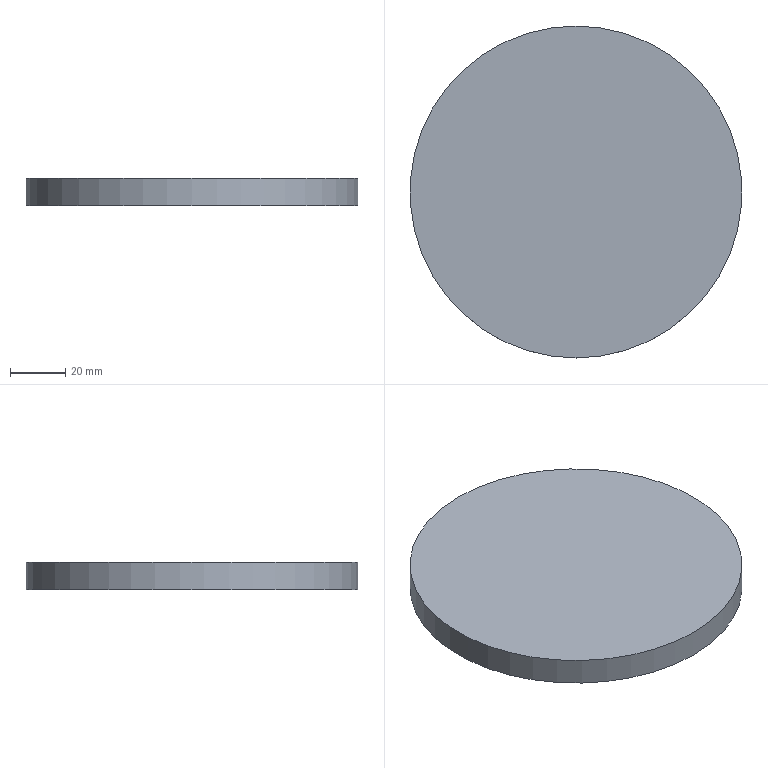Component | NX | CAM | 1 solid | 3 faces | box 120 x 120 x 10 mm | volume 113097 mm3 | plane 2 | cylinder 1 | commonest cylinder face diameters 120 x1
STEP:
#1=CARTESIAN_POINT('',(0.,0.,0.));
#2=DIRECTION('',(0.,0.,1.));
#3=DIRECTION('',(1.,0.,0.));
#4=AXIS2_PLACEMENT_3D('',#1,#2,#3);
#5=CARTESIAN_POINT('',(-1155.866,869.925,70.));
#6=VERTEX_POINT('',#5);
#7=CARTESIAN_POINT('',(-1155.866,809.925,70.));
#8=DIRECTION('',(0.,0.,1.));
#9=DIRECTION('',(0.,1.,0.));
#10=AXIS2_PLACEMENT_3D('',#7,#8,#9);
#11=CIRCLE('',#10,60.);
#12=CARTESIAN_POINT('',(-1155.866,809.925,70.));
#13=DIRECTION('',(0.,0.,-1.));
#14=DIRECTION('',(-1.,0.,0.));
#15=AXIS2_PLACEMENT_3D('',#12,#13,#14);
#16=CYLINDRICAL_SURFACE('',#15,60.);
#17=CARTESIAN_POINT('',(7.854,0.));
#18=DIRECTION('',(-1.,0.));
#19=VECTOR('',#18,1.);
#20=LINE('',#17,#19);
#21=(GEOMETRIC_REPRESENTATION_CONTEXT(2)PARAMETRIC_REPRESENTATION_CONTEXT()REPRESENTATION_CONTEXT('',''));
#22=DEFINITIONAL_REPRESENTATION('',(#20),#21);
#23=PCURVE('',#16,#22);
#24=CARTESIAN_POINT('',(-1155.866,809.925,70.));
#25=DIRECTION('',(0.,0.,1.));
#26=DIRECTION('',(1.,0.,0.));
#27=AXIS2_PLACEMENT_3D('',#24,#25,#26);
#28=PLANE('',#27);
#29=CARTESIAN_POINT('',(0.,0.));
#30=DIRECTION('',(0.,1.));
#31=AXIS2_PLACEMENT_2D('',#29,#30);
#32=CIRCLE('',#31,60.);
#33=(GEOMETRIC_REPRESENTATION_CONTEXT(2)PARAMETRIC_REPRESENTATION_CONTEXT()REPRESENTATION_CONTEXT('',''));
#34=DEFINITIONAL_REPRESENTATION('',(#32),#33);
#35=PCURVE('',#28,#34);
#36=SURFACE_CURVE('',#11,(#23,#35),.PCURVE_S1.);
#37=EDGE_CURVE('',#6,#6,#36,.T.);
#38=ORIENTED_EDGE('',*,*,#37,.F.);
#39=CARTESIAN_POINT('',(-1155.866,869.925,60.));
#40=VERTEX_POINT('',#39);
#41=CARTESIAN_POINT('',(-1155.866,869.925,70.));
#42=CARTESIAN_POINT('',(-1155.866,869.925,60.));
#43=B_SPLINE_CURVE_WITH_KNOTS('',1,(#41,#42),.UNSPECIFIED.,.F.,.F.,(2,2),(0.,10.),.PIECEWISE_BEZIER_KNOTS.);
#44=CARTESIAN_POINT('',(7.854,0.));
#45=DIRECTION('',(0.,1.));
#46=VECTOR('',#45,1.);
#47=LINE('',#44,#46);
#48=(GEOMETRIC_REPRESENTATION_CONTEXT(2)PARAMETRIC_REPRESENTATION_CONTEXT()REPRESENTATION_CONTEXT('',''));
#49=DEFINITIONAL_REPRESENTATION('',(#47),#48);
#50=PCURVE('',#16,#49);
#51=CARTESIAN_POINT('',(1.571,0.));
#52=DIRECTION('',(0.,1.));
#53=VECTOR('',#52,1.);
#54=LINE('',#51,#53);
#55=(GEOMETRIC_REPRESENTATION_CONTEXT(2)PARAMETRIC_REPRESENTATION_CONTEXT()REPRESENTATION_CONTEXT('',''));
#56=DEFINITIONAL_REPRESENTATION('',(#54),#55);
#57=PCURVE('',#16,#56);
#58=SEAM_CURVE('',#43,(#50,#57),.PCURVE_S1.);
#59=EDGE_CURVE('',#6,#40,#58,.T.);
#60=ORIENTED_EDGE('',*,*,#59,.T.);
#61=CARTESIAN_POINT('',(-1155.866,809.925,60.));
#62=DIRECTION('',(0.,0.,1.));
#63=DIRECTION('',(0.,1.,0.));
#64=AXIS2_PLACEMENT_3D('',#61,#62,#63);
#65=CIRCLE('',#64,60.);
#66=CARTESIAN_POINT('',(7.854,10.));
#67=DIRECTION('',(-1.,0.));
#68=VECTOR('',#67,1.);
#69=LINE('',#66,#68);
#70=(GEOMETRIC_REPRESENTATION_CONTEXT(2)PARAMETRIC_REPRESENTATION_CONTEXT()REPRESENTATION_CONTEXT('',''));
#71=DEFINITIONAL_REPRESENTATION('',(#69),#70);
#72=PCURVE('',#16,#71);
#73=CARTESIAN_POINT('',(-1155.866,809.925,60.));
#74=DIRECTION('',(0.,0.,1.));
#75=DIRECTION('',(1.,0.,0.));
#76=AXIS2_PLACEMENT_3D('',#73,#74,#75);
#77=PLANE('',#76);
#78=CARTESIAN_POINT('',(0.,0.));
#79=DIRECTION('',(0.,1.));
#80=AXIS2_PLACEMENT_2D('',#78,#79);
#81=CIRCLE('',#80,60.);
#82=(GEOMETRIC_REPRESENTATION_CONTEXT(2)PARAMETRIC_REPRESENTATION_CONTEXT()REPRESENTATION_CONTEXT('',''));
#83=DEFINITIONAL_REPRESENTATION('',(#81),#82);
#84=PCURVE('',#77,#83);
#85=SURFACE_CURVE('',#65,(#72,#84),.PCURVE_S1.);
#86=EDGE_CURVE('',#40,#40,#85,.T.);
#87=ORIENTED_EDGE('',*,*,#86,.T.);
#88=ORIENTED_EDGE('',*,*,#59,.F.);
#89=EDGE_LOOP('',(#38,#60,#87,#88));
#90=FACE_BOUND('',#89,.T.);
#91=ADVANCED_FACE('',(#90),#16,.T.);
#92=ORIENTED_EDGE('',*,*,#37,.T.);
#93=EDGE_LOOP('',(#92));
#94=FACE_BOUND('',#93,.T.);
#95=ADVANCED_FACE('',(#94),#28,.T.);
#96=ORIENTED_EDGE('',*,*,#86,.F.);
#97=EDGE_LOOP('',(#96));
#98=FACE_BOUND('',#97,.T.);
#99=ADVANCED_FACE('',(#98),#77,.F.);
#100=CLOSED_SHELL('',(#91,#95,#99));
#101=MANIFOLD_SOLID_BREP('',#100);
#102=(LENGTH_UNIT()NAMED_UNIT(*)SI_UNIT(.MILLI.,.METRE.));
#103=UNCERTAINTY_MEASURE_WITH_UNIT(LENGTH_MEASURE(0.00001),#102,'','');
#104=(NAMED_UNIT(*)PLANE_ANGLE_UNIT()SI_UNIT($,.RADIAN.));
#105=(NAMED_UNIT(*)SI_UNIT($,.STERADIAN.)SOLID_ANGLE_UNIT());
#106=(GEOMETRIC_REPRESENTATION_CONTEXT(3)GLOBAL_UNCERTAINTY_ASSIGNED_CONTEXT((#103))GLOBAL_UNIT_ASSIGNED_CONTEXT((#102,#104,#105))REPRESENTATION_CONTEXT('',''));
#107=ADVANCED_BREP_SHAPE_REPRESENTATION('',(#4,#101),#106);